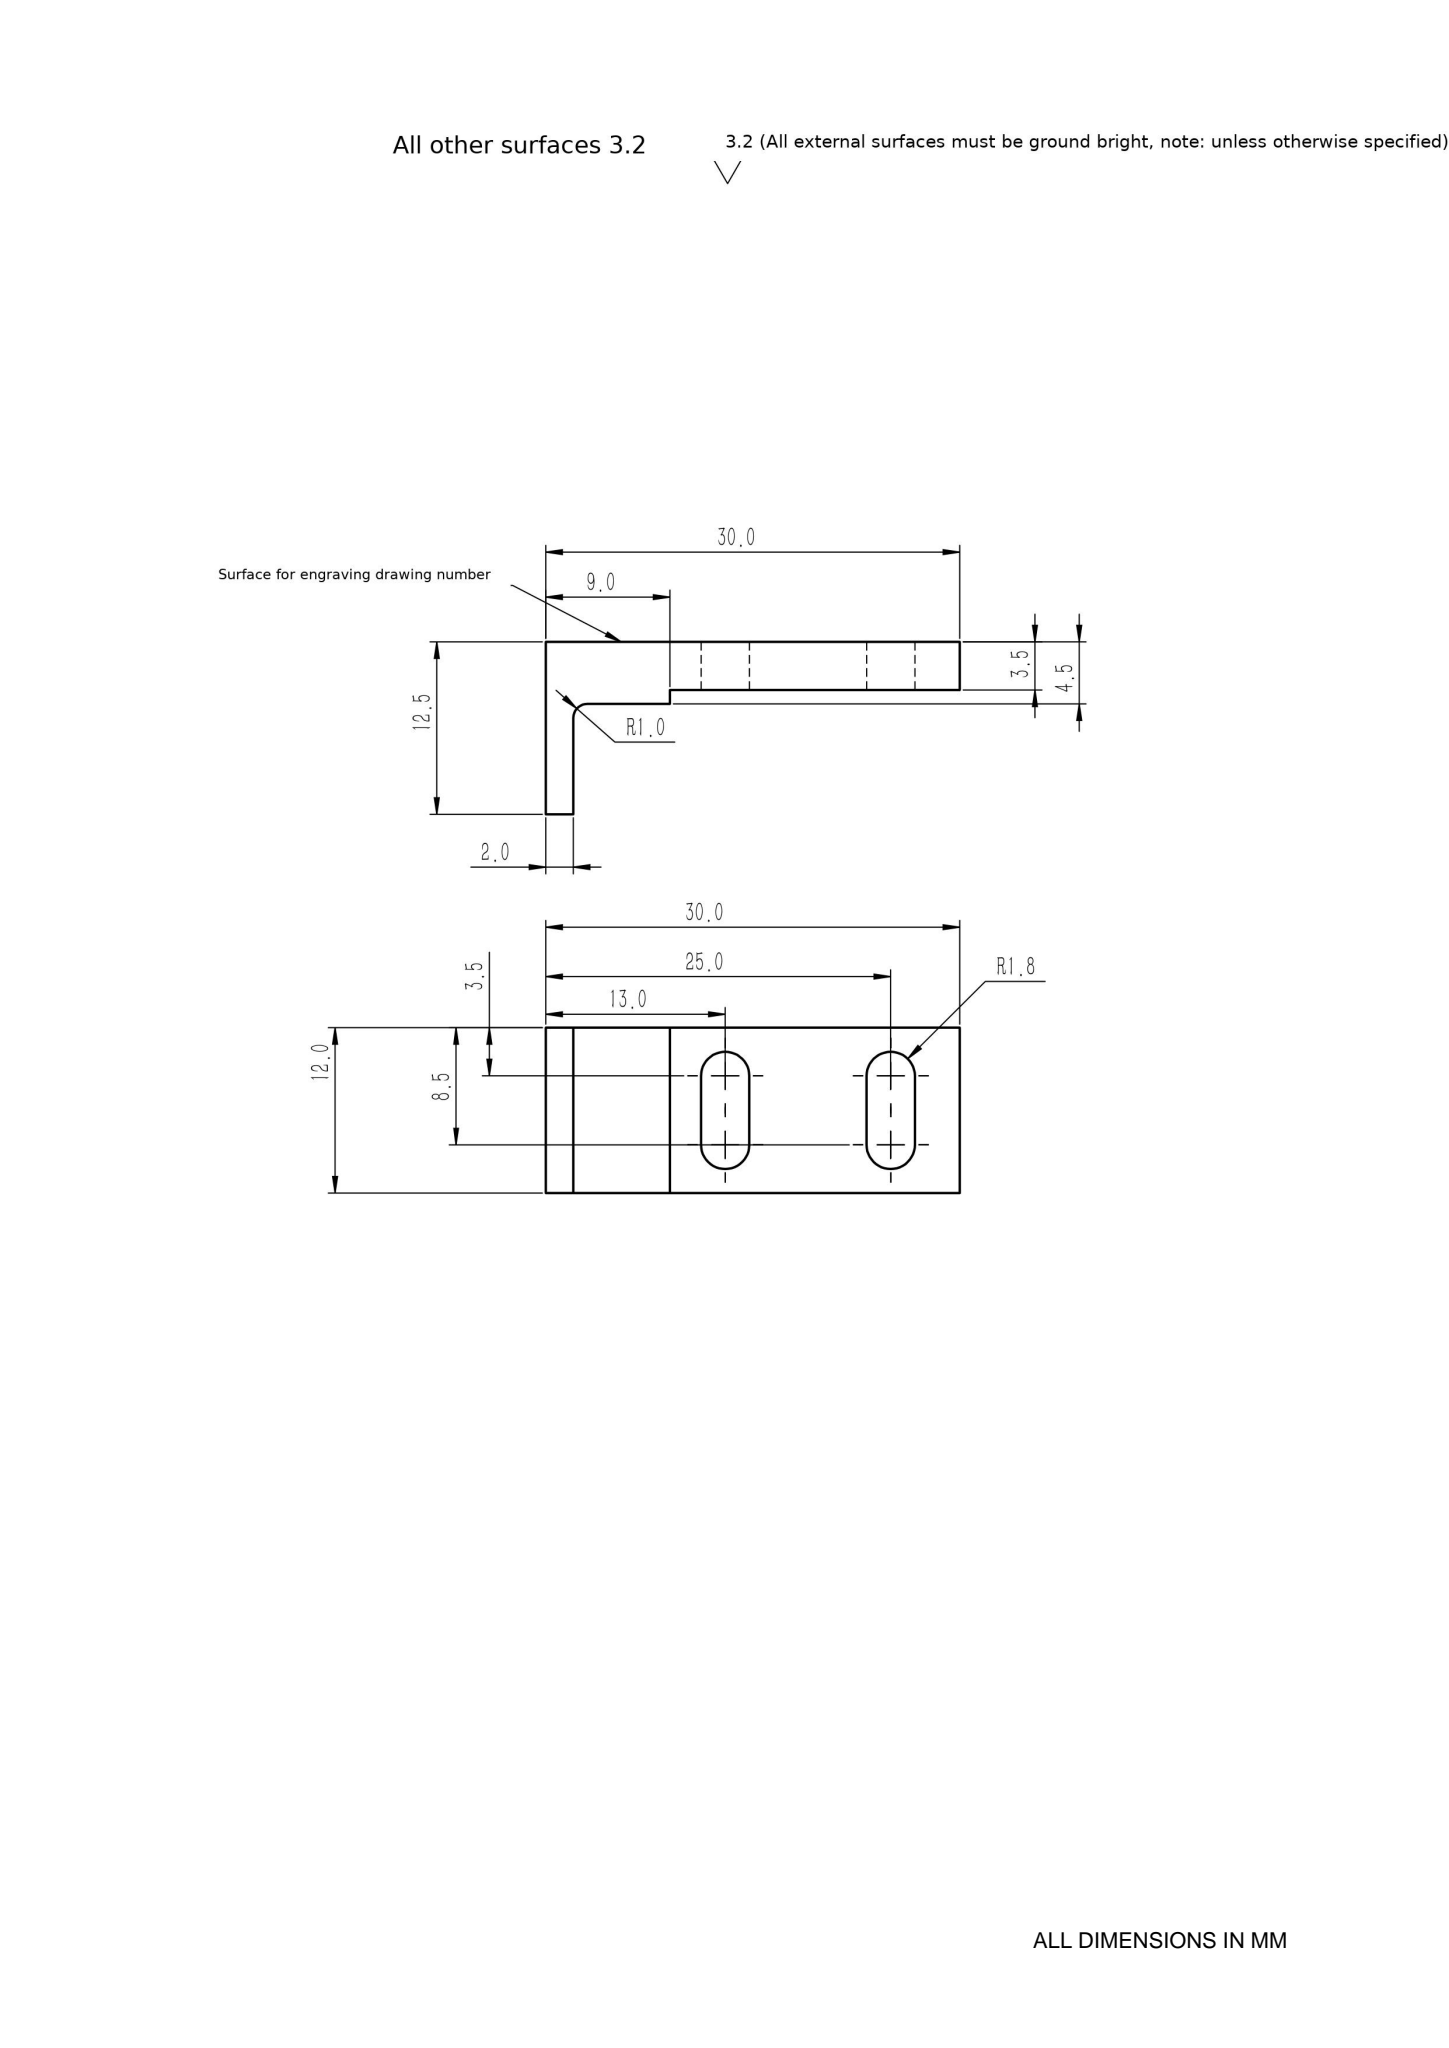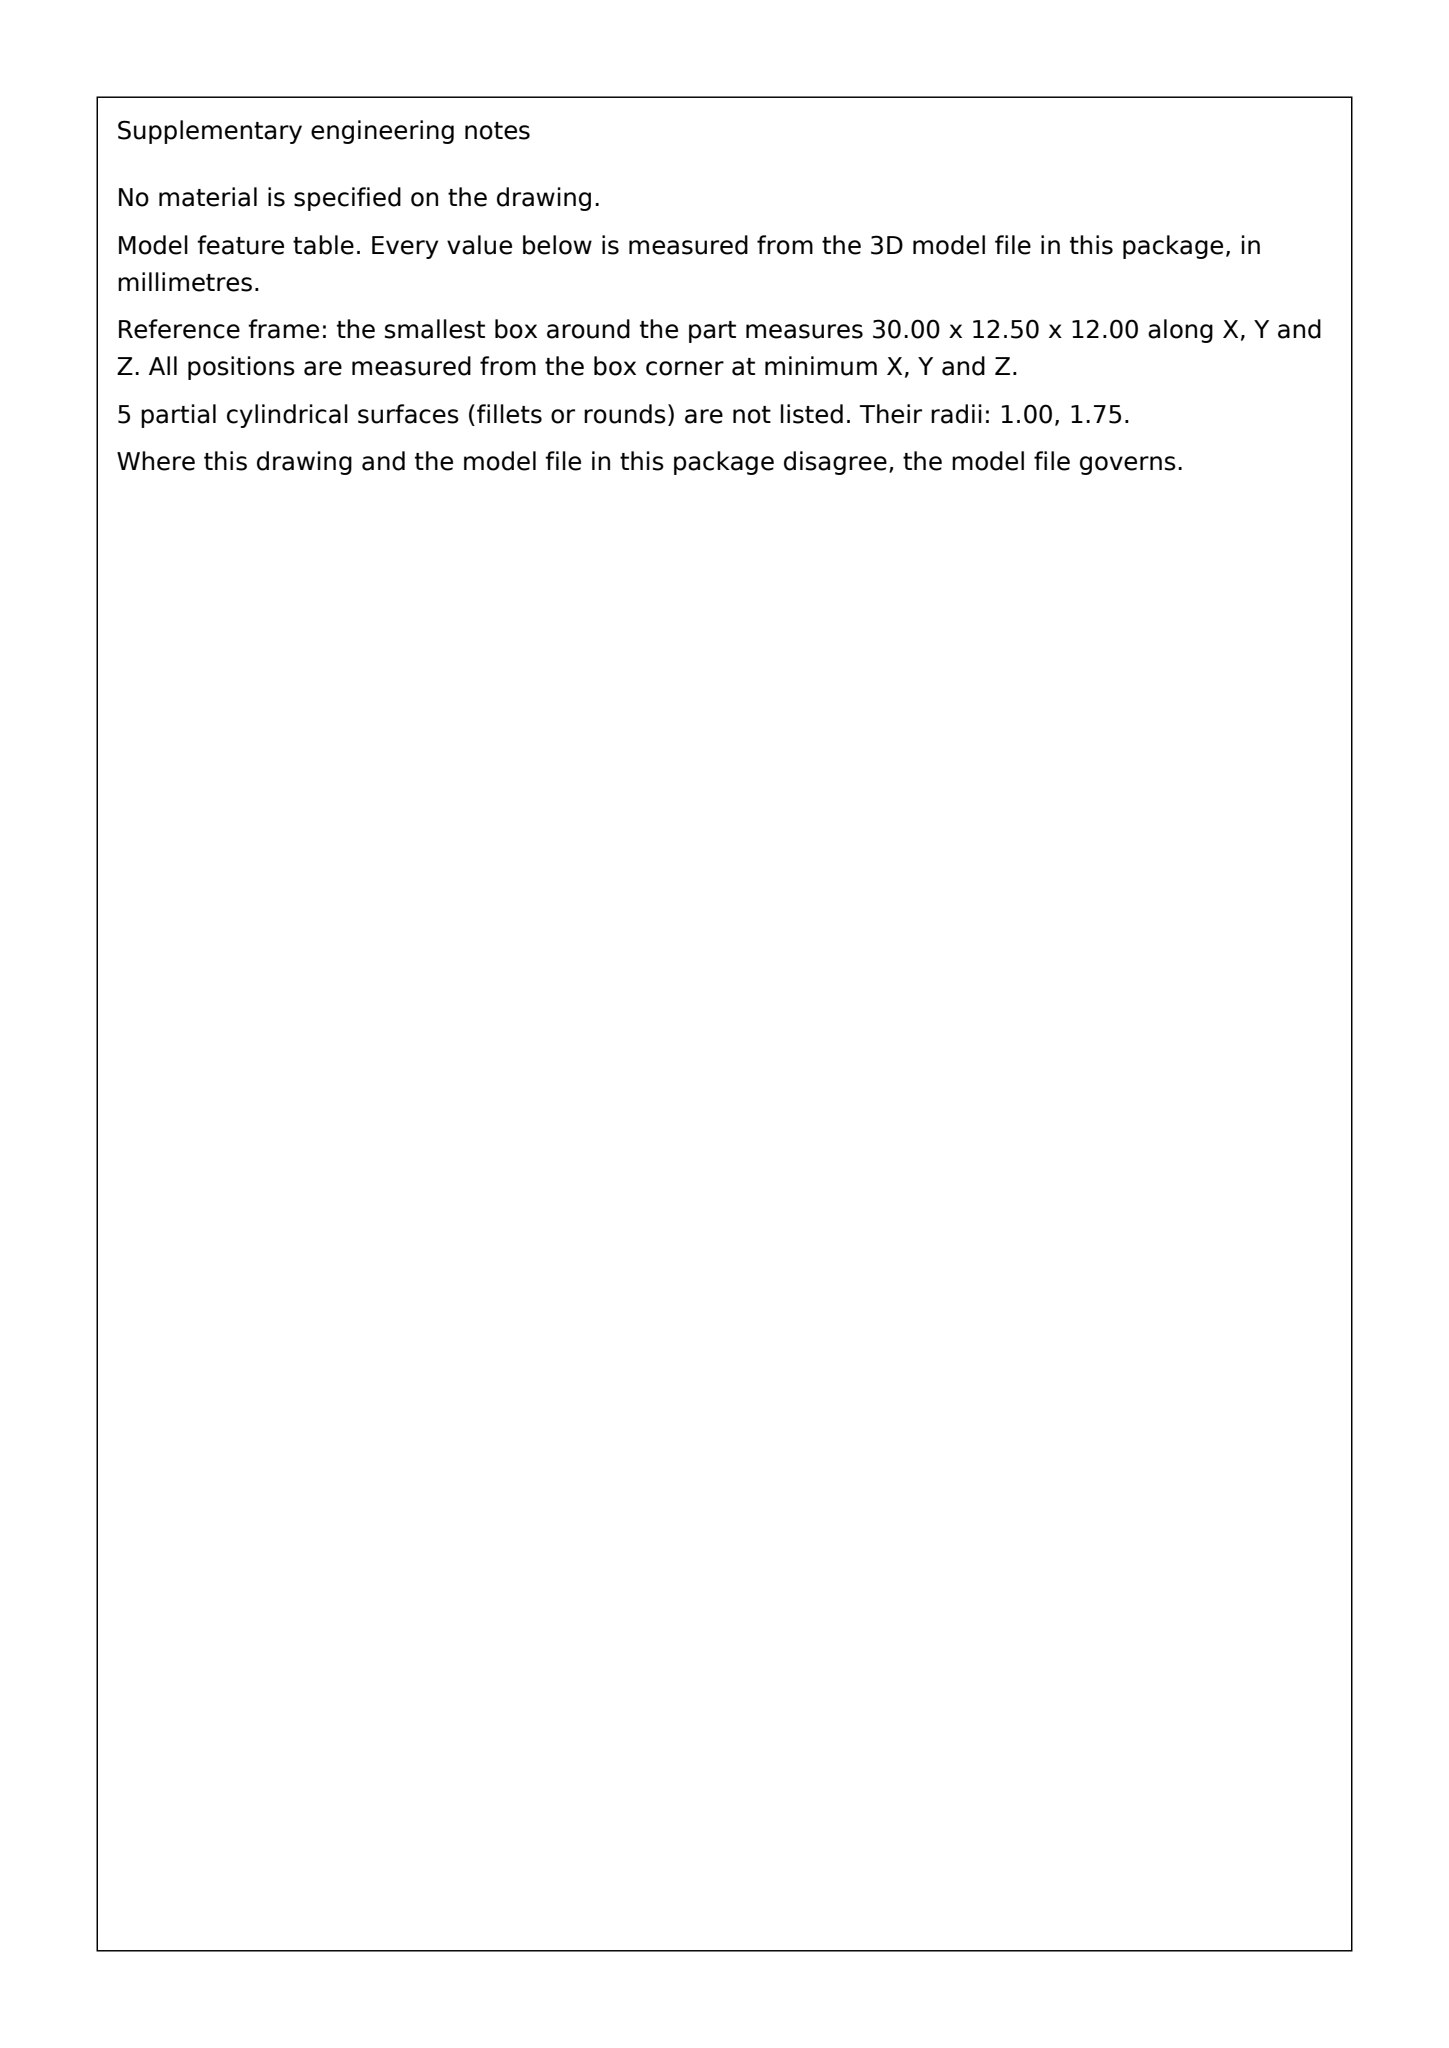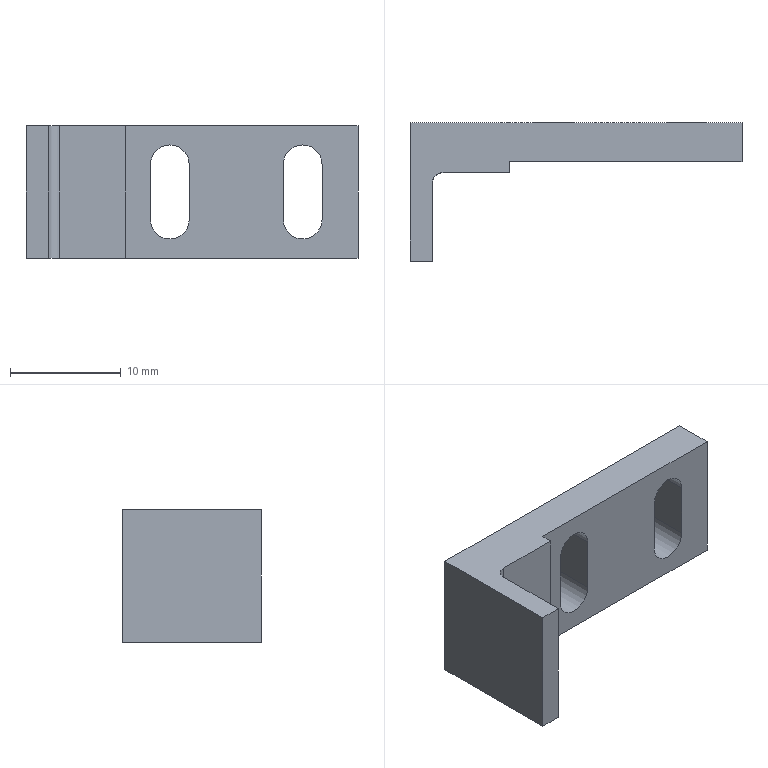Part | SolidWorks | mm | 1 solid | 21 faces | box 30 x 12.5 x 12 mm | volume 1373 mm3 | plane 14 | cylinder 7 | commonest cylinder face diameters 3.5 x6 2 x1
build123d program:
from build123d import *

# Parameters (mm, degrees)
EXTRUDE_THIN1_DEPTH = 12
LPATTERN1_COUNT     = 2
LPATTERN1_PITCH     = 12
BOSS_EXTRUDE1_START = 2.5
SKETCH4_W           = 30
SKETCH4_H           = 12
SKETCH4_R           = 1.7
BOSS_EXTRUDE1_DEPTH = 2.5
FILLET1_R           = 1
CUT_EXTRUDE1_DEPTH  = 10
SKETCH7_W           = 21
SKETCH7_H           = 12
CUT_EXTRUDE2_DEPTH  = 1


with BuildPart() as part:
    # Sketch1 → Extrude-Thin1 (new body)
    with BuildSketch(Plane.XY):
        Polygon((0, 0), (0, 10), (30, 10), (30, 8), (2, 8), (2, 0), align=None)
    extrude(amount=EXTRUDE_THIN1_DEPTH)

    # Sketch2 → 3.4 _3.4_ Diameter Hole1 (revolve, cut)
    with BuildSketch(Plane(origin=(25, 10, 4), x_dir=(0, 0, 1), z_dir=(1, 0, 0))):
        Polygon((0, 0), (0, 15.521), (1.7, 14.5), (1.7, 0), align=None)
    f_3_4_3_4_diameter_hole1 = revolve(axis=Axis((25, 16.35, 4), (0, -1, 0)), mode=Mode.SUBTRACT)

    # LPattern1: 3.4 _3.4_ Diameter Hole1 ×2
    with Locations(*[(-i * LPATTERN1_PITCH, 0, 0) for i in range(1, LPATTERN1_COUNT)]):
        add(f_3_4_3_4_diameter_hole1, mode=Mode.SUBTRACT)

    # Sketch4 → Boss-Extrude1 (add)
    with BuildSketch(Plane(origin=(0, 10, 0), x_dir=(1, 0, 0), z_dir=(0, 1, 0)).offset(BOSS_EXTRUDE1_START)):
        with Locations((15, -6)):
            Rectangle(SKETCH4_W, SKETCH4_H)
        with Locations(Location((13, -4, 0), (0, 0, 270))):
            Circle(SKETCH4_R, mode=Mode.SUBTRACT)
        with Locations(Location((25, -4, 0), (0, 0, 270))):
            Circle(SKETCH4_R, mode=Mode.SUBTRACT)
    extrude(amount=-BOSS_EXTRUDE1_DEPTH)

    # Fillet1
    fillet1_edges = [part.edges().sort_by_distance(p)[0] for p in [
        (2, 8, 6),
    ]]
    fillet(fillet1_edges, radius=FILLET1_R)

    # Sketch6 → Cut-Extrude1 (cut)
    with BuildSketch(Plane(origin=(0, 12.5, 0), x_dir=(1, 0, 0), z_dir=(0, 1, 0))):
        with BuildLine():
            Line((11.25, -8.5), (11.25, -3.5))
            ThreePointArc((11.25, -3.5), (13, -1.75), (14.75, -3.5))
            Line((14.75, -3.5), (14.75, -8.5))
            ThreePointArc((14.75, -8.5), (13, -10.25), (11.25, -8.5))
        make_face()
        with BuildLine():
            Line((26.75, -3.5), (26.75, -8.5))
            ThreePointArc((26.75, -8.5), (25, -10.25), (23.25, -8.5))
            Line((23.25, -8.5), (23.25, -3.5))
            ThreePointArc((23.25, -3.5), (25, -1.75), (26.75, -3.5))
        make_face()
    extrude(amount=-CUT_EXTRUDE1_DEPTH, mode=Mode.SUBTRACT)

    # Sketch7 → Cut-Extrude2 (cut)
    with BuildSketch(Plane.XZ.offset(-8)):
        with Locations((19.5, 6)):
            Rectangle(SKETCH7_W, SKETCH7_H)
    extrude(amount=-CUT_EXTRUDE2_DEPTH, mode=Mode.SUBTRACT)


solid = part.part
STEP:
#1=CARTESIAN_POINT('',(25.,9.,10.25));
#2=VERTEX_POINT('',#1);
#3=CARTESIAN_POINT('',(26.75,9.,8.5));
#4=VERTEX_POINT('',#3);
#5=CARTESIAN_POINT('',(25.,9.,8.5));
#6=DIRECTION('',(0.,1.,0.));
#7=DIRECTION('',(0.,0.,-1.));
#8=AXIS2_PLACEMENT_3D('',#5,#6,#7);
#9=CIRCLE('',#8,1.75);
#10=EDGE_CURVE('',#2,#4,#9,.T.);
#11=ORIENTED_EDGE('',*,*,#10,.F.);
#12=CARTESIAN_POINT('',(25.,12.5,10.25));
#13=VERTEX_POINT('',#12);
#14=CARTESIAN_POINT('',(25.,2.5,10.25));
#15=DIRECTION('',(0.,1.,0.));
#16=VECTOR('',#15,1000.);
#17=LINE('',#14,#16);
#18=EDGE_CURVE('',#2,#13,#17,.T.);
#19=ORIENTED_EDGE('',*,*,#18,.T.);
#20=CARTESIAN_POINT('',(26.75,12.5,8.5));
#21=VERTEX_POINT('',#20);
#22=CARTESIAN_POINT('',(25.,12.5,8.5));
#23=DIRECTION('',(0.,1.,0.));
#24=DIRECTION('',(0.,0.,1.));
#25=AXIS2_PLACEMENT_3D('',#22,#23,#24);
#26=CIRCLE('',#25,1.75);
#27=EDGE_CURVE('',#13,#21,#26,.T.);
#28=ORIENTED_EDGE('',*,*,#27,.T.);
#29=CARTESIAN_POINT('',(26.75,2.5,8.5));
#30=DIRECTION('',(0.,1.,0.));
#31=VECTOR('',#30,1000.);
#32=LINE('',#29,#31);
#33=EDGE_CURVE('',#4,#21,#32,.T.);
#34=ORIENTED_EDGE('',*,*,#33,.F.);
#35=EDGE_LOOP('',(#11,#19,#28,#34));
#36=FACE_OUTER_BOUND('',#35,.T.);
#37=CARTESIAN_POINT('',(25.,2.5,8.5));
#38=DIRECTION('',(0.,1.,0.));
#39=DIRECTION('',(0.,0.,1.));
#40=AXIS2_PLACEMENT_3D('',#37,#38,#39);
#41=CYLINDRICAL_SURFACE('',#40,1.75);
#42=ADVANCED_FACE('',(#36),#41,.F.);
#43=CARTESIAN_POINT('',(13.,9.,10.25));
#44=VERTEX_POINT('',#43);
#45=CARTESIAN_POINT('',(14.75,9.,8.5));
#46=VERTEX_POINT('',#45);
#47=CARTESIAN_POINT('',(13.,9.,8.5));
#48=DIRECTION('',(0.,1.,0.));
#49=DIRECTION('',(0.,0.,-1.));
#50=AXIS2_PLACEMENT_3D('',#47,#48,#49);
#51=CIRCLE('',#50,1.75);
#52=EDGE_CURVE('',#44,#46,#51,.T.);
#53=ORIENTED_EDGE('',*,*,#52,.F.);
#54=CARTESIAN_POINT('',(13.,12.5,10.25));
#55=VERTEX_POINT('',#54);
#56=CARTESIAN_POINT('',(13.,2.5,10.25));
#57=DIRECTION('',(0.,1.,0.));
#58=VECTOR('',#57,1000.);
#59=LINE('',#56,#58);
#60=EDGE_CURVE('',#44,#55,#59,.T.);
#61=ORIENTED_EDGE('',*,*,#60,.T.);
#62=CARTESIAN_POINT('',(14.75,12.5,8.5));
#63=VERTEX_POINT('',#62);
#64=CARTESIAN_POINT('',(13.,12.5,8.5));
#65=DIRECTION('',(0.,1.,0.));
#66=DIRECTION('',(0.,0.,1.));
#67=AXIS2_PLACEMENT_3D('',#64,#65,#66);
#68=CIRCLE('',#67,1.75);
#69=EDGE_CURVE('',#55,#63,#68,.T.);
#70=ORIENTED_EDGE('',*,*,#69,.T.);
#71=CARTESIAN_POINT('',(14.75,2.5,8.5));
#72=DIRECTION('',(0.,1.,0.));
#73=VECTOR('',#72,1000.);
#74=LINE('',#71,#73);
#75=EDGE_CURVE('',#46,#63,#74,.T.);
#76=ORIENTED_EDGE('',*,*,#75,.F.);
#77=EDGE_LOOP('',(#53,#61,#70,#76));
#78=FACE_OUTER_BOUND('',#77,.T.);
#79=CARTESIAN_POINT('',(13.,2.5,8.5));
#80=DIRECTION('',(0.,1.,0.));
#81=DIRECTION('',(0.,0.,1.));
#82=AXIS2_PLACEMENT_3D('',#79,#80,#81);
#83=CYLINDRICAL_SURFACE('',#82,1.75);
#84=ADVANCED_FACE('',(#78),#83,.F.);
#85=CARTESIAN_POINT('',(30.,12.5,12.));
#86=VERTEX_POINT('',#85);
#87=CARTESIAN_POINT('',(30.,9.,12.));
#88=VERTEX_POINT('',#87);
#89=CARTESIAN_POINT('',(30.,10.,12.));
#90=DIRECTION('',(0.,-1.,0.));
#91=VECTOR('',#90,1000.);
#92=LINE('',#89,#91);
#93=EDGE_CURVE('',#86,#88,#92,.T.);
#94=ORIENTED_EDGE('',*,*,#93,.T.);
#95=CARTESIAN_POINT('',(30.,9.,0.));
#96=VERTEX_POINT('',#95);
#97=CARTESIAN_POINT('',(30.,9.,12.));
#98=DIRECTION('',(0.,0.,1.));
#99=VECTOR('',#98,1000.);
#100=LINE('',#97,#99);
#101=EDGE_CURVE('',#96,#88,#100,.T.);
#102=ORIENTED_EDGE('',*,*,#101,.F.);
#103=CARTESIAN_POINT('',(30.,12.5,0.));
#104=VERTEX_POINT('',#103);
#105=CARTESIAN_POINT('',(30.,10.,0.));
#106=DIRECTION('',(0.,-1.,0.));
#107=VECTOR('',#106,1000.);
#108=LINE('',#105,#107);
#109=EDGE_CURVE('',#104,#96,#108,.T.);
#110=ORIENTED_EDGE('',*,*,#109,.F.);
#111=CARTESIAN_POINT('',(30.,12.5,12.));
#112=DIRECTION('',(0.,0.,-1.));
#113=VECTOR('',#112,1000.);
#114=LINE('',#111,#113);
#115=EDGE_CURVE('',#86,#104,#114,.T.);
#116=ORIENTED_EDGE('',*,*,#115,.F.);
#117=EDGE_LOOP('',(#94,#102,#110,#116));
#118=FACE_OUTER_BOUND('',#117,.T.);
#119=CARTESIAN_POINT('',(30.,10.,12.));
#120=DIRECTION('',(1.,0.,0.));
#121=DIRECTION('',(0.,0.,-1.));
#122=AXIS2_PLACEMENT_3D('',#119,#120,#121);
#123=PLANE('',#122);
#124=ADVANCED_FACE('',(#118),#123,.T.);
#125=ORIENTED_EDGE('',*,*,#60,.F.);
#126=CARTESIAN_POINT('',(11.25,9.,8.5));
#127=VERTEX_POINT('',#126);
#128=CARTESIAN_POINT('',(13.,9.,8.5));
#129=DIRECTION('',(0.,1.,0.));
#130=DIRECTION('',(0.,0.,-1.));
#131=AXIS2_PLACEMENT_3D('',#128,#129,#130);
#132=CIRCLE('',#131,1.75);
#133=EDGE_CURVE('',#127,#44,#132,.T.);
#134=ORIENTED_EDGE('',*,*,#133,.F.);
#135=CARTESIAN_POINT('',(11.25,12.5,8.5));
#136=VERTEX_POINT('',#135);
#137=CARTESIAN_POINT('',(11.25,2.5,8.5));
#138=DIRECTION('',(0.,1.,0.));
#139=VECTOR('',#138,1000.);
#140=LINE('',#137,#139);
#141=EDGE_CURVE('',#127,#136,#140,.T.);
#142=ORIENTED_EDGE('',*,*,#141,.T.);
#143=CARTESIAN_POINT('',(13.,12.5,8.5));
#144=DIRECTION('',(0.,1.,0.));
#145=DIRECTION('',(0.,0.,1.));
#146=AXIS2_PLACEMENT_3D('',#143,#144,#145);
#147=CIRCLE('',#146,1.75);
#148=EDGE_CURVE('',#136,#55,#147,.T.);
#149=ORIENTED_EDGE('',*,*,#148,.T.);
#150=EDGE_LOOP('',(#125,#134,#142,#149));
#151=FACE_OUTER_BOUND('',#150,.T.);
#152=CARTESIAN_POINT('',(13.,2.5,8.5));
#153=DIRECTION('',(0.,1.,0.));
#154=DIRECTION('',(0.,0.,1.));
#155=AXIS2_PLACEMENT_3D('',#152,#153,#154);
#156=CYLINDRICAL_SURFACE('',#155,1.75);
#157=ADVANCED_FACE('',(#151),#156,.F.);
#158=CARTESIAN_POINT('',(11.25,9.,3.5));
#159=VERTEX_POINT('',#158);
#160=CARTESIAN_POINT('',(11.25,9.,8.5));
#161=DIRECTION('',(0.,0.,1.));
#162=VECTOR('',#161,1000.);
#163=LINE('',#160,#162);
#164=EDGE_CURVE('',#159,#127,#163,.T.);
#165=ORIENTED_EDGE('',*,*,#164,.F.);
#166=CARTESIAN_POINT('',(11.25,12.5,3.5));
#167=VERTEX_POINT('',#166);
#168=CARTESIAN_POINT('',(11.25,2.5,3.5));
#169=DIRECTION('',(0.,1.,0.));
#170=VECTOR('',#169,1000.);
#171=LINE('',#168,#170);
#172=EDGE_CURVE('',#159,#167,#171,.T.);
#173=ORIENTED_EDGE('',*,*,#172,.T.);
#174=CARTESIAN_POINT('',(11.25,12.5,8.5));
#175=DIRECTION('',(0.,0.,1.));
#176=VECTOR('',#175,1000.);
#177=LINE('',#174,#176);
#178=EDGE_CURVE('',#167,#136,#177,.T.);
#179=ORIENTED_EDGE('',*,*,#178,.T.);
#180=ORIENTED_EDGE('',*,*,#141,.F.);
#181=EDGE_LOOP('',(#165,#173,#179,#180));
#182=FACE_OUTER_BOUND('',#181,.T.);
#183=CARTESIAN_POINT('',(11.25,2.5,8.5));
#184=DIRECTION('',(-1.,0.,0.));
#185=DIRECTION('',(0.,0.,1.));
#186=AXIS2_PLACEMENT_3D('',#183,#184,#185);
#187=PLANE('',#186);
#188=ADVANCED_FACE('',(#182),#187,.F.);
#189=CARTESIAN_POINT('',(14.75,9.,3.5));
#190=VERTEX_POINT('',#189);
#191=CARTESIAN_POINT('',(13.,9.,3.5));
#192=DIRECTION('',(0.,1.,0.));
#193=DIRECTION('',(0.,0.,-1.));
#194=AXIS2_PLACEMENT_3D('',#191,#192,#193);
#195=CIRCLE('',#194,1.75);
#196=EDGE_CURVE('',#190,#159,#195,.T.);
#197=ORIENTED_EDGE('',*,*,#196,.F.);
#198=CARTESIAN_POINT('',(14.75,12.5,3.5));
#199=VERTEX_POINT('',#198);
#200=CARTESIAN_POINT('',(14.75,2.5,3.5));
#201=DIRECTION('',(0.,1.,0.));
#202=VECTOR('',#201,1000.);
#203=LINE('',#200,#202);
#204=EDGE_CURVE('',#190,#199,#203,.T.);
#205=ORIENTED_EDGE('',*,*,#204,.T.);
#206=CARTESIAN_POINT('',(13.,12.5,3.5));
#207=DIRECTION('',(0.,1.,0.));
#208=DIRECTION('',(0.,0.,1.));
#209=AXIS2_PLACEMENT_3D('',#206,#207,#208);
#210=CIRCLE('',#209,1.75);
#211=EDGE_CURVE('',#199,#167,#210,.T.);
#212=ORIENTED_EDGE('',*,*,#211,.T.);
#213=ORIENTED_EDGE('',*,*,#172,.F.);
#214=EDGE_LOOP('',(#197,#205,#212,#213));
#215=FACE_OUTER_BOUND('',#214,.T.);
#216=CARTESIAN_POINT('',(13.,2.5,3.5));
#217=DIRECTION('',(0.,1.,0.));
#218=DIRECTION('',(0.,0.,1.));
#219=AXIS2_PLACEMENT_3D('',#216,#217,#218);
#220=CYLINDRICAL_SURFACE('',#219,1.75);
#221=ADVANCED_FACE('',(#215),#220,.F.);
#222=CARTESIAN_POINT('',(14.75,9.,8.5));
#223=DIRECTION('',(0.,0.,-1.));
#224=VECTOR('',#223,1000.);
#225=LINE('',#222,#224);
#226=EDGE_CURVE('',#46,#190,#225,.T.);
#227=ORIENTED_EDGE('',*,*,#226,.F.);
#228=ORIENTED_EDGE('',*,*,#75,.T.);
#229=CARTESIAN_POINT('',(14.75,12.5,8.5));
#230=DIRECTION('',(0.,0.,-1.));
#231=VECTOR('',#230,1000.);
#232=LINE('',#229,#231);
#233=EDGE_CURVE('',#63,#199,#232,.T.);
#234=ORIENTED_EDGE('',*,*,#233,.T.);
#235=ORIENTED_EDGE('',*,*,#204,.F.);
#236=EDGE_LOOP('',(#227,#228,#234,#235));
#237=FACE_OUTER_BOUND('',#236,.T.);
#238=CARTESIAN_POINT('',(14.75,2.5,8.5));
#239=DIRECTION('',(1.,0.,0.));
#240=DIRECTION('',(0.,0.,-1.));
#241=AXIS2_PLACEMENT_3D('',#238,#239,#240);
#242=PLANE('',#241);
#243=ADVANCED_FACE('',(#237),#242,.F.);
#244=CARTESIAN_POINT('',(26.75,9.,3.5));
#245=VERTEX_POINT('',#244);
#246=CARTESIAN_POINT('',(23.25,9.,3.5));
#247=VERTEX_POINT('',#246);
#248=CARTESIAN_POINT('',(25.,9.,3.5));
#249=DIRECTION('',(0.,1.,0.));
#250=DIRECTION('',(0.,0.,-1.));
#251=AXIS2_PLACEMENT_3D('',#248,#249,#250);
#252=CIRCLE('',#251,1.75);
#253=EDGE_CURVE('',#245,#247,#252,.T.);
#254=ORIENTED_EDGE('',*,*,#253,.F.);
#255=CARTESIAN_POINT('',(26.75,12.5,3.5));
#256=VERTEX_POINT('',#255);
#257=CARTESIAN_POINT('',(26.75,2.5,3.5));
#258=DIRECTION('',(0.,1.,0.));
#259=VECTOR('',#258,1000.);
#260=LINE('',#257,#259);
#261=EDGE_CURVE('',#245,#256,#260,.T.);
#262=ORIENTED_EDGE('',*,*,#261,.T.);
#263=CARTESIAN_POINT('',(23.25,12.5,3.5));
#264=VERTEX_POINT('',#263);
#265=CARTESIAN_POINT('',(25.,12.5,3.5));
#266=DIRECTION('',(0.,1.,0.));
#267=DIRECTION('',(0.,0.,1.));
#268=AXIS2_PLACEMENT_3D('',#265,#266,#267);
#269=CIRCLE('',#268,1.75);
#270=EDGE_CURVE('',#256,#264,#269,.T.);
#271=ORIENTED_EDGE('',*,*,#270,.T.);
#272=CARTESIAN_POINT('',(23.25,2.5,3.5));
#273=DIRECTION('',(0.,1.,0.));
#274=VECTOR('',#273,1000.);
#275=LINE('',#272,#274);
#276=EDGE_CURVE('',#247,#264,#275,.T.);
#277=ORIENTED_EDGE('',*,*,#276,.F.);
#278=EDGE_LOOP('',(#254,#262,#271,#277));
#279=FACE_OUTER_BOUND('',#278,.T.);
#280=CARTESIAN_POINT('',(25.,2.5,3.5));
#281=DIRECTION('',(0.,1.,0.));
#282=DIRECTION('',(0.,0.,1.));
#283=AXIS2_PLACEMENT_3D('',#280,#281,#282);
#284=CYLINDRICAL_SURFACE('',#283,1.75);
#285=ADVANCED_FACE('',(#279),#284,.F.);
#286=CARTESIAN_POINT('',(26.75,9.,3.5));
#287=DIRECTION('',(0.,0.,-1.));
#288=VECTOR('',#287,1000.);
#289=LINE('',#286,#288);
#290=EDGE_CURVE('',#4,#245,#289,.T.);
#291=ORIENTED_EDGE('',*,*,#290,.F.);
#292=ORIENTED_EDGE('',*,*,#33,.T.);
#293=CARTESIAN_POINT('',(26.75,12.5,3.5));
#294=DIRECTION('',(0.,0.,-1.));
#295=VECTOR('',#294,1000.);
#296=LINE('',#293,#295);
#297=EDGE_CURVE('',#21,#256,#296,.T.);
#298=ORIENTED_EDGE('',*,*,#297,.T.);
#299=ORIENTED_EDGE('',*,*,#261,.F.);
#300=EDGE_LOOP('',(#291,#292,#298,#299));
#301=FACE_OUTER_BOUND('',#300,.T.);
#302=CARTESIAN_POINT('',(26.75,2.5,3.5));
#303=DIRECTION('',(1.,0.,0.));
#304=DIRECTION('',(0.,0.,-1.));
#305=AXIS2_PLACEMENT_3D('',#302,#303,#304);
#306=PLANE('',#305);
#307=ADVANCED_FACE('',(#301),#306,.F.);
#308=ORIENTED_EDGE('',*,*,#18,.F.);
#309=CARTESIAN_POINT('',(23.25,9.,8.5));
#310=VERTEX_POINT('',#309);
#311=CARTESIAN_POINT('',(25.,9.,8.5));
#312=DIRECTION('',(0.,1.,0.));
#313=DIRECTION('',(0.,0.,-1.));
#314=AXIS2_PLACEMENT_3D('',#311,#312,#313);
#315=CIRCLE('',#314,1.75);
#316=EDGE_CURVE('',#310,#2,#315,.T.);
#317=ORIENTED_EDGE('',*,*,#316,.F.);
#318=CARTESIAN_POINT('',(23.25,12.5,8.5));
#319=VERTEX_POINT('',#318);
#320=CARTESIAN_POINT('',(23.25,2.5,8.5));
#321=DIRECTION('',(0.,1.,0.));
#322=VECTOR('',#321,1000.);
#323=LINE('',#320,#322);
#324=EDGE_CURVE('',#310,#319,#323,.T.);
#325=ORIENTED_EDGE('',*,*,#324,.T.);
#326=CARTESIAN_POINT('',(25.,12.5,8.5));
#327=DIRECTION('',(0.,1.,0.));
#328=DIRECTION('',(0.,0.,1.));
#329=AXIS2_PLACEMENT_3D('',#326,#327,#328);
#330=CIRCLE('',#329,1.75);
#331=EDGE_CURVE('',#319,#13,#330,.T.);
#332=ORIENTED_EDGE('',*,*,#331,.T.);
#333=EDGE_LOOP('',(#308,#317,#325,#332));
#334=FACE_OUTER_BOUND('',#333,.T.);
#335=CARTESIAN_POINT('',(25.,2.5,8.5));
#336=DIRECTION('',(0.,1.,0.));
#337=DIRECTION('',(0.,0.,1.));
#338=AXIS2_PLACEMENT_3D('',#335,#336,#337);
#339=CYLINDRICAL_SURFACE('',#338,1.75);
#340=ADVANCED_FACE('',(#334),#339,.F.);
#341=CARTESIAN_POINT('',(23.25,9.,3.5));
#342=DIRECTION('',(0.,0.,1.));
#343=VECTOR('',#342,1000.);
#344=LINE('',#341,#343);
#345=EDGE_CURVE('',#247,#310,#344,.T.);
#346=ORIENTED_EDGE('',*,*,#345,.F.);
#347=ORIENTED_EDGE('',*,*,#276,.T.);
#348=CARTESIAN_POINT('',(23.25,12.5,3.5));
#349=DIRECTION('',(0.,0.,1.));
#350=VECTOR('',#349,1000.);
#351=LINE('',#348,#350);
#352=EDGE_CURVE('',#264,#319,#351,.T.);
#353=ORIENTED_EDGE('',*,*,#352,.T.);
#354=ORIENTED_EDGE('',*,*,#324,.F.);
#355=EDGE_LOOP('',(#346,#347,#353,#354));
#356=FACE_OUTER_BOUND('',#355,.T.);
#357=CARTESIAN_POINT('',(23.25,2.5,3.5));
#358=DIRECTION('',(-1.,0.,0.));
#359=DIRECTION('',(0.,0.,1.));
#360=AXIS2_PLACEMENT_3D('',#357,#358,#359);
#361=PLANE('',#360);
#362=ADVANCED_FACE('',(#356),#361,.F.);
#363=CARTESIAN_POINT('',(3.,8.,0.));
#364=VERTEX_POINT('',#363);
#365=CARTESIAN_POINT('',(9.,8.,0.));
#366=VERTEX_POINT('',#365);
#367=CARTESIAN_POINT('',(0.,8.,0.));
#368=DIRECTION('',(1.,0.,0.));
#369=VECTOR('',#368,1000.);
#370=LINE('',#367,#369);
#371=EDGE_CURVE('',#364,#366,#370,.T.);
#372=ORIENTED_EDGE('',*,*,#371,.T.);
#373=CARTESIAN_POINT('',(9.,8.,12.));
#374=VERTEX_POINT('',#373);
#375=CARTESIAN_POINT('',(9.,8.,12.));
#376=DIRECTION('',(0.,0.,-1.));
#377=VECTOR('',#376,1000.);
#378=LINE('',#375,#377);
#379=EDGE_CURVE('',#374,#366,#378,.T.);
#380=ORIENTED_EDGE('',*,*,#379,.F.);
#381=CARTESIAN_POINT('',(3.,8.,12.));
#382=VERTEX_POINT('',#381);
#383=CARTESIAN_POINT('',(0.,8.,12.));
#384=DIRECTION('',(1.,0.,0.));
#385=VECTOR('',#384,1000.);
#386=LINE('',#383,#385);
#387=EDGE_CURVE('',#382,#374,#386,.T.);
#388=ORIENTED_EDGE('',*,*,#387,.F.);
#389=CARTESIAN_POINT('',(3.,8.,0.));
#390=DIRECTION('',(0.,0.,-1.));
#391=VECTOR('',#390,1000.);
#392=LINE('',#389,#391);
#393=EDGE_CURVE('',#382,#364,#392,.T.);
#394=ORIENTED_EDGE('',*,*,#393,.T.);
#395=EDGE_LOOP('',(#372,#380,#388,#394));
#396=FACE_OUTER_BOUND('',#395,.T.);
#397=CARTESIAN_POINT('',(0.,8.,12.));
#398=DIRECTION('',(0.,1.,0.));
#399=DIRECTION('',(0.,0.,1.));
#400=AXIS2_PLACEMENT_3D('',#397,#398,#399);
#401=PLANE('',#400);
#402=ADVANCED_FACE('',(#396),#401,.F.);
#403=CARTESIAN_POINT('',(0.,0.,0.));
#404=VERTEX_POINT('',#403);
#405=CARTESIAN_POINT('',(0.,12.5,0.));
#406=VERTEX_POINT('',#405);
#407=CARTESIAN_POINT('',(0.,0.,0.));
#408=DIRECTION('',(0.,1.,0.));
#409=VECTOR('',#408,1000.);
#410=LINE('',#407,#409);
#411=EDGE_CURVE('',#404,#406,#410,.T.);
#412=ORIENTED_EDGE('',*,*,#411,.F.);
#413=CARTESIAN_POINT('',(0.,0.,12.));
#414=VERTEX_POINT('',#413);
#415=CARTESIAN_POINT('',(0.,0.,12.));
#416=DIRECTION('',(0.,0.,-1.));
#417=VECTOR('',#416,1000.);
#418=LINE('',#415,#417);
#419=EDGE_CURVE('',#414,#404,#418,.T.);
#420=ORIENTED_EDGE('',*,*,#419,.F.);
#421=CARTESIAN_POINT('',(0.,12.5,12.));
#422=VERTEX_POINT('',#421);
#423=CARTESIAN_POINT('',(0.,0.,12.));
#424=DIRECTION('',(0.,1.,0.));
#425=VECTOR('',#424,1000.);
#426=LINE('',#423,#425);
#427=EDGE_CURVE('',#414,#422,#426,.T.);
#428=ORIENTED_EDGE('',*,*,#427,.T.);
#429=CARTESIAN_POINT('',(0.,12.5,0.));
#430=DIRECTION('',(0.,0.,1.));
#431=VECTOR('',#430,1000.);
#432=LINE('',#429,#431);
#433=EDGE_CURVE('',#406,#422,#432,.T.);
#434=ORIENTED_EDGE('',*,*,#433,.F.);
#435=EDGE_LOOP('',(#412,#420,#428,#434));
#436=FACE_OUTER_BOUND('',#435,.T.);
#437=CARTESIAN_POINT('',(0.,0.,12.));
#438=DIRECTION('',(-1.,0.,0.));
#439=DIRECTION('',(0.,0.,1.));
#440=AXIS2_PLACEMENT_3D('',#437,#438,#439);
#441=PLANE('',#440);
#442=ADVANCED_FACE('',(#436),#441,.T.);
#443=CARTESIAN_POINT('',(2.,0.,0.));
#444=VERTEX_POINT('',#443);
#445=CARTESIAN_POINT('',(2.,0.,0.));
#446=DIRECTION('',(-1.,0.,0.));
#447=VECTOR('',#446,1000.);
#448=LINE('',#445,#447);
#449=EDGE_CURVE('',#444,#404,#448,.T.);
#450=ORIENTED_EDGE('',*,*,#449,.F.);
#451=CARTESIAN_POINT('',(2.,0.,12.));
#452=VERTEX_POINT('',#451);
#453=CARTESIAN_POINT('',(2.,0.,12.));
#454=DIRECTION('',(0.,0.,-1.));
#455=VECTOR('',#454,1000.);
#456=LINE('',#453,#455);
#457=EDGE_CURVE('',#452,#444,#456,.T.);
#458=ORIENTED_EDGE('',*,*,#457,.F.);
#459=CARTESIAN_POINT('',(2.,0.,12.));
#460=DIRECTION('',(-1.,0.,0.));
#461=VECTOR('',#460,1000.);
#462=LINE('',#459,#461);
#463=EDGE_CURVE('',#452,#414,#462,.T.);
#464=ORIENTED_EDGE('',*,*,#463,.T.);
#465=ORIENTED_EDGE('',*,*,#419,.T.);
#466=EDGE_LOOP('',(#450,#458,#464,#465));
#467=FACE_OUTER_BOUND('',#466,.T.);
#468=CARTESIAN_POINT('',(2.,0.,12.));
#469=DIRECTION('',(0.,-1.,0.));
#470=DIRECTION('',(0.,0.,-1.));
#471=AXIS2_PLACEMENT_3D('',#468,#469,#470);
#472=PLANE('',#471);
#473=ADVANCED_FACE('',(#467),#472,.T.);
#474=CARTESIAN_POINT('',(2.,7.,0.));
#475=VERTEX_POINT('',#474);
#476=CARTESIAN_POINT('',(2.,0.,0.));
#477=DIRECTION('',(0.,1.,0.));
#478=VECTOR('',#477,1000.);
#479=LINE('',#476,#478);
#480=EDGE_CURVE('',#444,#475,#479,.T.);
#481=ORIENTED_EDGE('',*,*,#480,.T.);
#482=CARTESIAN_POINT('',(2.,7.,12.));
#483=VERTEX_POINT('',#482);
#484=CARTESIAN_POINT('',(2.,7.,12.));
#485=DIRECTION('',(0.,0.,1.));
#486=VECTOR('',#485,1000.);
#487=LINE('',#484,#486);
#488=EDGE_CURVE('',#475,#483,#487,.T.);
#489=ORIENTED_EDGE('',*,*,#488,.T.);
#490=CARTESIAN_POINT('',(2.,0.,12.));
#491=DIRECTION('',(0.,1.,0.));
#492=VECTOR('',#491,1000.);
#493=LINE('',#490,#492);
#494=EDGE_CURVE('',#452,#483,#493,.T.);
#495=ORIENTED_EDGE('',*,*,#494,.F.);
#496=ORIENTED_EDGE('',*,*,#457,.T.);
#497=EDGE_LOOP('',(#481,#489,#495,#496));
#498=FACE_OUTER_BOUND('',#497,.T.);
#499=CARTESIAN_POINT('',(2.,0.,12.));
#500=DIRECTION('',(-1.,0.,0.));
#501=DIRECTION('',(0.,0.,1.));
#502=AXIS2_PLACEMENT_3D('',#499,#500,#501);
#503=PLANE('',#502);
#504=ADVANCED_FACE('',(#498),#503,.F.);
#505=ORIENTED_EDGE('',*,*,#387,.T.);
#506=CARTESIAN_POINT('',(9.,9.,12.));
#507=VERTEX_POINT('',#506);
#508=CARTESIAN_POINT('',(9.,9.,12.));
#509=DIRECTION('',(0.,-1.,0.));
#510=VECTOR('',#509,1000.);
#511=LINE('',#508,#510);
#512=EDGE_CURVE('',#507,#374,#511,.T.);
#513=ORIENTED_EDGE('',*,*,#512,.F.);
#514=CARTESIAN_POINT('',(9.,9.,12.));
#515=DIRECTION('',(-1.,0.,0.));
#516=VECTOR('',#515,1000.);
#517=LINE('',#514,#516);
#518=EDGE_CURVE('',#88,#507,#517,.T.);
#519=ORIENTED_EDGE('',*,*,#518,.F.);
#520=ORIENTED_EDGE('',*,*,#93,.F.);
#521=CARTESIAN_POINT('',(0.,12.5,12.));
#522=DIRECTION('',(1.,0.,0.));
#523=VECTOR('',#522,1000.);
#524=LINE('',#521,#523);
#525=EDGE_CURVE('',#422,#86,#524,.T.);
#526=ORIENTED_EDGE('',*,*,#525,.F.);
#527=ORIENTED_EDGE('',*,*,#427,.F.);
#528=ORIENTED_EDGE('',*,*,#463,.F.);
#529=ORIENTED_EDGE('',*,*,#494,.T.);
#530=CARTESIAN_POINT('',(3.,7.,12.));
#531=DIRECTION('',(0.,0.,-1.));
#532=DIRECTION('',(-1.,0.,0.));
#533=AXIS2_PLACEMENT_3D('',#530,#531,#532);
#534=CIRCLE('',#533,1.);
#535=EDGE_CURVE('',#483,#382,#534,.T.);
#536=ORIENTED_EDGE('',*,*,#535,.T.);
#537=EDGE_LOOP('',(#505,#513,#519,#520,#526,#527,#528,#529,#536));
#538=FACE_OUTER_BOUND('',#537,.T.);
#539=CARTESIAN_POINT('',(0.,0.,12.));
#540=DIRECTION('',(0.,0.,-1.));
#541=DIRECTION('',(-1.,0.,0.));
#542=AXIS2_PLACEMENT_3D('',#539,#540,#541);
#543=PLANE('',#542);
#544=ADVANCED_FACE('',(#538),#543,.F.);
#545=CARTESIAN_POINT('',(9.,9.,0.));
#546=VERTEX_POINT('',#545);
#547=CARTESIAN_POINT('',(9.,9.,0.));
#548=DIRECTION('',(0.,-1.,0.));
#549=VECTOR('',#548,1000.);
#550=LINE('',#547,#549);
#551=EDGE_CURVE('',#546,#366,#550,.T.);
#552=ORIENTED_EDGE('',*,*,#551,.T.);
#553=ORIENTED_EDGE('',*,*,#371,.F.);
#554=CARTESIAN_POINT('',(3.,7.,0.));
#555=DIRECTION('',(0.,0.,1.));
#556=DIRECTION('',(-1.,0.,0.));
#557=AXIS2_PLACEMENT_3D('',#554,#555,#556);
#558=CIRCLE('',#557,1.);
#559=EDGE_CURVE('',#364,#475,#558,.T.);
#560=ORIENTED_EDGE('',*,*,#559,.T.);
#561=ORIENTED_EDGE('',*,*,#480,.F.);
#562=ORIENTED_EDGE('',*,*,#449,.T.);
#563=ORIENTED_EDGE('',*,*,#411,.T.);
#564=CARTESIAN_POINT('',(30.,12.5,0.));
#565=DIRECTION('',(-1.,0.,0.));
#566=VECTOR('',#565,1000.);
#567=LINE('',#564,#566);
#568=EDGE_CURVE('',#104,#406,#567,.T.);
#569=ORIENTED_EDGE('',*,*,#568,.F.);
#570=ORIENTED_EDGE('',*,*,#109,.T.);
#571=CARTESIAN_POINT('',(9.,9.,0.));
#572=DIRECTION('',(1.,0.,0.));
#573=VECTOR('',#572,1000.);
#574=LINE('',#571,#573);
#575=EDGE_CURVE('',#546,#96,#574,.T.);
#576=ORIENTED_EDGE('',*,*,#575,.F.);
#577=EDGE_LOOP('',(#552,#553,#560,#561,#562,#563,#569,#570,#576));
#578=FACE_OUTER_BOUND('',#577,.T.);
#579=CARTESIAN_POINT('',(0.,0.,0.));
#580=DIRECTION('',(0.,0.,-1.));
#581=DIRECTION('',(-1.,0.,0.));
#582=AXIS2_PLACEMENT_3D('',#579,#580,#581);
#583=PLANE('',#582);
#584=ADVANCED_FACE('',(#578),#583,.T.);
#585=ORIENTED_EDGE('',*,*,#270,.F.);
#586=ORIENTED_EDGE('',*,*,#297,.F.);
#587=ORIENTED_EDGE('',*,*,#27,.F.);
#588=ORIENTED_EDGE('',*,*,#331,.F.);
#589=ORIENTED_EDGE('',*,*,#352,.F.);
#590=EDGE_LOOP('',(#585,#586,#587,#588,#589));
#591=FACE_BOUND('',#590,.T.);
#592=ORIENTED_EDGE('',*,*,#148,.F.);
#593=ORIENTED_EDGE('',*,*,#178,.F.);
#594=ORIENTED_EDGE('',*,*,#211,.F.);
#595=ORIENTED_EDGE('',*,*,#233,.F.);
#596=ORIENTED_EDGE('',*,*,#69,.F.);
#597=EDGE_LOOP('',(#592,#593,#594,#595,#596));
#598=FACE_BOUND('',#597,.T.);
#599=ORIENTED_EDGE('',*,*,#115,.T.);
#600=ORIENTED_EDGE('',*,*,#568,.T.);
#601=ORIENTED_EDGE('',*,*,#433,.T.);
#602=ORIENTED_EDGE('',*,*,#525,.T.);
#603=EDGE_LOOP('',(#599,#600,#601,#602));
#604=FACE_OUTER_BOUND('',#603,.T.);
#605=CARTESIAN_POINT('',(0.,12.5,0.));
#606=DIRECTION('',(0.,1.,0.));
#607=DIRECTION('',(0.,0.,1.));
#608=AXIS2_PLACEMENT_3D('',#605,#606,#607);
#609=PLANE('',#608);
#610=ADVANCED_FACE('',(#591,#598,#604),#609,.T.);
#611=ORIENTED_EDGE('',*,*,#535,.F.);
#612=ORIENTED_EDGE('',*,*,#488,.F.);
#613=ORIENTED_EDGE('',*,*,#559,.F.);
#614=ORIENTED_EDGE('',*,*,#393,.F.);
#615=EDGE_LOOP('',(#611,#612,#613,#614));
#616=FACE_OUTER_BOUND('',#615,.T.);
#617=CARTESIAN_POINT('',(3.,7.,12.));
#618=DIRECTION('',(0.,0.,1.));
#619=DIRECTION('',(1.,0.,0.));
#620=AXIS2_PLACEMENT_3D('',#617,#618,#619);
#621=CYLINDRICAL_SURFACE('',#620,1.);
#622=ADVANCED_FACE('',(#616),#621,.F.);
#623=ORIENTED_EDGE('',*,*,#253,.T.);
#624=ORIENTED_EDGE('',*,*,#345,.T.);
#625=ORIENTED_EDGE('',*,*,#316,.T.);
#626=ORIENTED_EDGE('',*,*,#10,.T.);
#627=ORIENTED_EDGE('',*,*,#290,.T.);
#628=EDGE_LOOP('',(#623,#624,#625,#626,#627));
#629=FACE_BOUND('',#628,.T.);
#630=ORIENTED_EDGE('',*,*,#101,.T.);
#631=ORIENTED_EDGE('',*,*,#518,.T.);
#632=CARTESIAN_POINT('',(9.,9.,12.));
#633=DIRECTION('',(0.,0.,-1.));
#634=VECTOR('',#633,1000.);
#635=LINE('',#632,#634);
#636=EDGE_CURVE('',#507,#546,#635,.T.);
#637=ORIENTED_EDGE('',*,*,#636,.T.);
#638=ORIENTED_EDGE('',*,*,#575,.T.);
#639=EDGE_LOOP('',(#630,#631,#637,#638));
#640=FACE_OUTER_BOUND('',#639,.T.);
#641=ORIENTED_EDGE('',*,*,#133,.T.);
#642=ORIENTED_EDGE('',*,*,#52,.T.);
#643=ORIENTED_EDGE('',*,*,#226,.T.);
#644=ORIENTED_EDGE('',*,*,#196,.T.);
#645=ORIENTED_EDGE('',*,*,#164,.T.);
#646=EDGE_LOOP('',(#641,#642,#643,#644,#645));
#647=FACE_BOUND('',#646,.T.);
#648=CARTESIAN_POINT('',(0.,9.,0.));
#649=DIRECTION('',(0.,-1.,0.));
#650=DIRECTION('',(0.,0.,-1.));
#651=AXIS2_PLACEMENT_3D('',#648,#649,#650);
#652=PLANE('',#651);
#653=ADVANCED_FACE('',(#629,#640,#647),#652,.T.);
#654=ORIENTED_EDGE('',*,*,#379,.T.);
#655=ORIENTED_EDGE('',*,*,#551,.F.);
#656=ORIENTED_EDGE('',*,*,#636,.F.);
#657=ORIENTED_EDGE('',*,*,#512,.T.);
#658=EDGE_LOOP('',(#654,#655,#656,#657));
#659=FACE_OUTER_BOUND('',#658,.T.);
#660=CARTESIAN_POINT('',(9.,9.,12.));
#661=DIRECTION('',(-1.,0.,-0.));
#662=DIRECTION('',(-0.,0.,1.));
#663=AXIS2_PLACEMENT_3D('',#660,#661,#662);
#664=PLANE('',#663);
#665=ADVANCED_FACE('',(#659),#664,.F.);
#666=CLOSED_SHELL('',(#42,#84,#124,#157,#188,#221,#243,#285,#307,#340,#362,#402,#442,#473,#504,#544,#584,#610,#622,#653,#665));
#667=MANIFOLD_SOLID_BREP('',#666);
#668=CARTESIAN_POINT('',(0.,0.,0.));
#669=DIRECTION('',(0.,0.,1.));
#670=DIRECTION('',(1.,0.,0.));
#671=AXIS2_PLACEMENT_3D('',#668,#669,#670);
#672=(LENGTH_UNIT()NAMED_UNIT(*)SI_UNIT(.MILLI.,.METRE.));
#673=UNCERTAINTY_MEASURE_WITH_UNIT(LENGTH_MEASURE(0.00001),#672,'','');
#674=(NAMED_UNIT(*)PLANE_ANGLE_UNIT()SI_UNIT($,.RADIAN.));
#675=(NAMED_UNIT(*)SI_UNIT($,.STERADIAN.)SOLID_ANGLE_UNIT());
#676=(GEOMETRIC_REPRESENTATION_CONTEXT(3)GLOBAL_UNCERTAINTY_ASSIGNED_CONTEXT((#673))GLOBAL_UNIT_ASSIGNED_CONTEXT((#672,#674,#675))REPRESENTATION_CONTEXT('',''));
#677=ADVANCED_BREP_SHAPE_REPRESENTATION('',(#667,#671),#676);